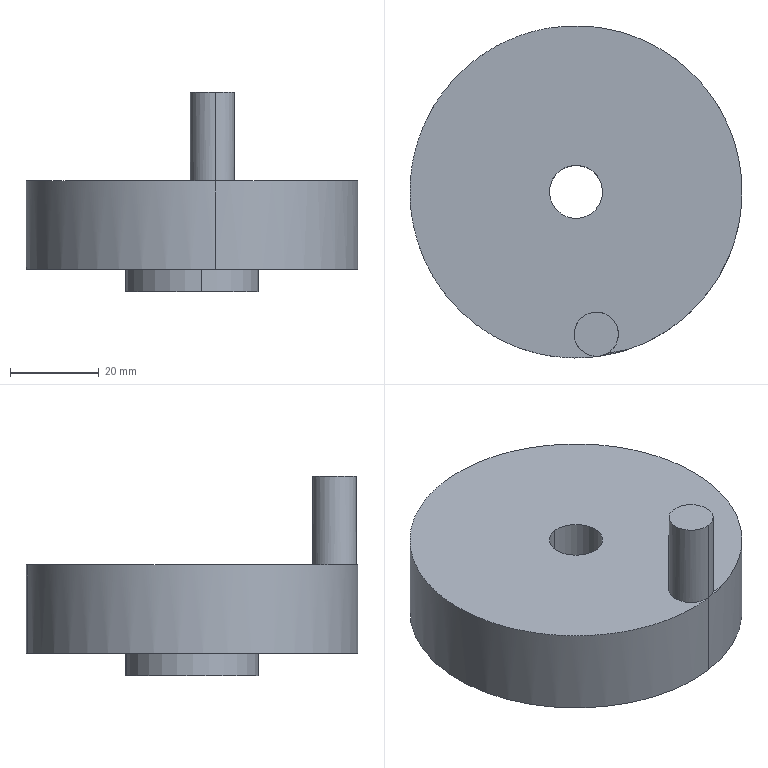Component | SolidWorks | Turntable-2 | 1 solid | 12 faces | box 75 x 75 x 45 mm | volume 90635 mm3 | cylinder 8 | plane 4 | commonest cylinder face diameters 30 x2 10 x2 12 x2 75 x2
build123d program:
from build123d import *

# Parameters (mm, degrees)
SKETCH1_R           = 37.5
SKETCH1_R_2         = 6
BOSS_EXTRUDE1_DEPTH = 20
SKETCH2_R           = 5
BOSS_EXTRUDE2_DEPTH = 20
SKETCH3_R           = 15
SKETCH3_R_2         = 6
BOSS_EXTRUDE3_DEPTH = 5


with BuildPart() as part:
    # Sketch1 → Boss-Extrude1 (new body)
    with BuildSketch(Plane.XY):
        with Locations((-30, 0)):
            Circle(SKETCH1_R)
        with Locations((-30, 0)):
            Circle(SKETCH1_R_2, mode=Mode.SUBTRACT)
    extrude(amount=-BOSS_EXTRUDE1_DEPTH)

    # Sketch2 → Boss-Extrude2 (add)
    with BuildSketch(Plane.XY):
        with Locations((2.5, 0)):
            Circle(SKETCH2_R)
    extrude(amount=BOSS_EXTRUDE2_DEPTH)

    # Sketch3 → Boss-Extrude3 (add)
    with BuildSketch(Plane(origin=(0, 0, -20), x_dir=(-1, 0, 0), z_dir=(0, 0, -1))):
        with Locations(Location((30, 0, 0), (0, 0, 180))):
            Circle(SKETCH3_R)
        with Locations(Location((30, 0, 0), (0, 0, 180))):
            Circle(SKETCH3_R_2, mode=Mode.SUBTRACT)
    extrude(amount=BOSS_EXTRUDE3_DEPTH)


solid = part.part

# Placed as in the assembly
solid = solid.moved(Location((-65.143, -96.872, 127.182), (0, 0, -81.89)))
STEP:
#1=COLOUR_RGB('',0.7922,0.8196,0.9333);
#2=FILL_AREA_STYLE_COLOUR('',#1);
#3=FILL_AREA_STYLE('',(#2));
#4=SURFACE_STYLE_FILL_AREA(#3);
#5=SURFACE_SIDE_STYLE('',(#4));
#6=SURFACE_STYLE_USAGE(.BOTH.,#5);
#7=PRESENTATION_STYLE_ASSIGNMENT((#6));
#8=CARTESIAN_POINT('',(-2.815,-2.06,4.023));
#9=VERTEX_POINT('',#8);
#10=CARTESIAN_POINT('',(-2.648,-3.229,4.023));
#11=VERTEX_POINT('',#10);
#12=CARTESIAN_POINT('',(-2.731,-2.645,4.023));
#13=DIRECTION('',(0.,-0.,-1.));
#14=DIRECTION('',(-0.1411,0.99,0.));
#15=AXIS2_PLACEMENT_3D('',#12,#13,#14);
#16=CIRCLE('',#15,0.5906);
#17=EDGE_CURVE('',#9,#11,#16,.T.);
#18=ORIENTED_EDGE('',*,*,#17,.F.);
#19=CARTESIAN_POINT('',(-2.815,-2.06,4.22));
#20=VERTEX_POINT('',#19);
#21=CARTESIAN_POINT('',(-2.815,-2.06,4.023));
#22=DIRECTION('',(-0.,0.,1.));
#23=VECTOR('',#22,39.37);
#24=LINE('',#21,#23);
#25=EDGE_CURVE('',#9,#20,#24,.T.);
#26=ORIENTED_EDGE('',*,*,#25,.T.);
#27=CARTESIAN_POINT('',(-2.648,-3.229,4.22));
#28=VERTEX_POINT('',#27);
#29=CARTESIAN_POINT('',(-2.731,-2.645,4.22));
#30=DIRECTION('',(0.,-0.,-1.));
#31=DIRECTION('',(0.1411,-0.99,0.));
#32=AXIS2_PLACEMENT_3D('',#29,#30,#31);
#33=CIRCLE('',#32,0.5906);
#34=EDGE_CURVE('',#20,#28,#33,.T.);
#35=ORIENTED_EDGE('',*,*,#34,.T.);
#36=CARTESIAN_POINT('',(-2.648,-3.229,4.023));
#37=DIRECTION('',(-0.,0.,1.));
#38=VECTOR('',#37,39.37);
#39=LINE('',#36,#38);
#40=EDGE_CURVE('',#11,#28,#39,.T.);
#41=ORIENTED_EDGE('',*,*,#40,.F.);
#42=EDGE_LOOP('',(#18,#26,#35,#41));
#43=FACE_OUTER_BOUND('',#42,.T.);
#44=CARTESIAN_POINT('',(-2.731,-2.645,4.023));
#45=DIRECTION('',(-0.,0.,1.));
#46=DIRECTION('',(0.1411,-0.99,0.));
#47=AXIS2_PLACEMENT_3D('',#44,#45,#46);
#48=CYLINDRICAL_SURFACE('',#47,0.5906);
#49=ADVANCED_FACE('',(#43),#48,.T.);
#50=CARTESIAN_POINT('',(-2.523,-4.106,5.795));
#51=VERTEX_POINT('',#50);
#52=CARTESIAN_POINT('',(-2.579,-3.716,5.795));
#53=VERTEX_POINT('',#52);
#54=CARTESIAN_POINT('',(-2.551,-3.911,5.795));
#55=DIRECTION('',(-0.,0.,1.));
#56=DIRECTION('',(0.1411,-0.99,0.));
#57=AXIS2_PLACEMENT_3D('',#54,#55,#56);
#58=CIRCLE('',#57,0.1969);
#59=EDGE_CURVE('',#51,#53,#58,.T.);
#60=ORIENTED_EDGE('',*,*,#59,.F.);
#61=CARTESIAN_POINT('',(-2.523,-4.106,5.007));
#62=VERTEX_POINT('',#61);
#63=CARTESIAN_POINT('',(-2.523,-4.106,5.795));
#64=DIRECTION('',(0.,-0.,-1.));
#65=VECTOR('',#64,39.37);
#66=LINE('',#63,#65);
#67=EDGE_CURVE('',#51,#62,#66,.T.);
#68=ORIENTED_EDGE('',*,*,#67,.T.);
#69=CARTESIAN_POINT('',(-2.579,-3.716,5.007));
#70=VERTEX_POINT('',#69);
#71=CARTESIAN_POINT('',(-2.551,-3.911,5.007));
#72=DIRECTION('',(-0.,0.,1.));
#73=DIRECTION('',(0.1411,-0.99,0.));
#74=AXIS2_PLACEMENT_3D('',#71,#72,#73);
#75=CIRCLE('',#74,0.1969);
#76=EDGE_CURVE('',#62,#70,#75,.T.);
#77=ORIENTED_EDGE('',*,*,#76,.T.);
#78=CARTESIAN_POINT('',(-2.579,-3.716,5.795));
#79=DIRECTION('',(0.,-0.,-1.));
#80=VECTOR('',#79,39.37);
#81=LINE('',#78,#80);
#82=EDGE_CURVE('',#53,#70,#81,.T.);
#83=ORIENTED_EDGE('',*,*,#82,.F.);
#84=EDGE_LOOP('',(#60,#68,#77,#83));
#85=FACE_OUTER_BOUND('',#84,.T.);
#86=CARTESIAN_POINT('',(-2.551,-3.911,5.795));
#87=DIRECTION('',(0.,-0.,-1.));
#88=DIRECTION('',(-0.1411,0.99,0.));
#89=AXIS2_PLACEMENT_3D('',#86,#87,#88);
#90=CYLINDRICAL_SURFACE('',#89,0.1969);
#91=ADVANCED_FACE('',(#85),#90,.T.);
#92=CARTESIAN_POINT('',(-2.698,-2.878,4.023));
#93=VERTEX_POINT('',#92);
#94=CARTESIAN_POINT('',(-2.765,-2.411,4.023));
#95=VERTEX_POINT('',#94);
#96=CARTESIAN_POINT('',(-2.731,-2.645,4.023));
#97=DIRECTION('',(0.,-0.,-1.));
#98=DIRECTION('',(-0.1411,0.99,0.));
#99=AXIS2_PLACEMENT_3D('',#96,#97,#98);
#100=CIRCLE('',#99,0.2362);
#101=EDGE_CURVE('',#93,#95,#100,.T.);
#102=ORIENTED_EDGE('',*,*,#101,.T.);
#103=CARTESIAN_POINT('',(-2.765,-2.411,5.007));
#104=VERTEX_POINT('',#103);
#105=CARTESIAN_POINT('',(-2.765,-2.411,4.22));
#106=DIRECTION('',(-0.,0.,1.));
#107=VECTOR('',#106,39.37);
#108=LINE('',#105,#107);
#109=EDGE_CURVE('',#95,#104,#108,.T.);
#110=ORIENTED_EDGE('',*,*,#109,.T.);
#111=CARTESIAN_POINT('',(-2.698,-2.878,5.007));
#112=VERTEX_POINT('',#111);
#113=CARTESIAN_POINT('',(-2.731,-2.645,5.007));
#114=DIRECTION('',(-0.,0.,1.));
#115=DIRECTION('',(0.1411,-0.99,0.));
#116=AXIS2_PLACEMENT_3D('',#113,#114,#115);
#117=CIRCLE('',#116,0.2362);
#118=EDGE_CURVE('',#104,#112,#117,.T.);
#119=ORIENTED_EDGE('',*,*,#118,.T.);
#120=CARTESIAN_POINT('',(-2.698,-2.878,4.22));
#121=DIRECTION('',(-0.,0.,1.));
#122=VECTOR('',#121,39.37);
#123=LINE('',#120,#122);
#124=EDGE_CURVE('',#93,#112,#123,.T.);
#125=ORIENTED_EDGE('',*,*,#124,.F.);
#126=EDGE_LOOP('',(#102,#110,#119,#125));
#127=FACE_OUTER_BOUND('',#126,.T.);
#128=CARTESIAN_POINT('',(-2.731,-2.645,4.22));
#129=DIRECTION('',(-0.,0.,1.));
#130=DIRECTION('',(0.1411,-0.99,0.));
#131=AXIS2_PLACEMENT_3D('',#128,#129,#130);
#132=CYLINDRICAL_SURFACE('',#131,0.2362);
#133=ADVANCED_FACE('',(#127),#132,.F.);
#134=CARTESIAN_POINT('',(-2.523,-4.106,4.22));
#135=VERTEX_POINT('',#134);
#136=CARTESIAN_POINT('',(-2.94,-1.183,4.22));
#137=VERTEX_POINT('',#136);
#138=CARTESIAN_POINT('',(-2.731,-2.645,4.22));
#139=DIRECTION('',(-0.,0.,1.));
#140=DIRECTION('',(0.1411,-0.99,0.));
#141=AXIS2_PLACEMENT_3D('',#138,#139,#140);
#142=CIRCLE('',#141,1.476);
#143=EDGE_CURVE('',#135,#137,#142,.T.);
#144=ORIENTED_EDGE('',*,*,#143,.T.);
#145=CARTESIAN_POINT('',(-2.94,-1.183,5.007));
#146=VERTEX_POINT('',#145);
#147=CARTESIAN_POINT('',(-2.94,-1.183,4.22));
#148=DIRECTION('',(-0.,0.,1.));
#149=VECTOR('',#148,39.37);
#150=LINE('',#147,#149);
#151=EDGE_CURVE('',#137,#146,#150,.T.);
#152=ORIENTED_EDGE('',*,*,#151,.T.);
#153=CARTESIAN_POINT('',(-2.731,-2.645,5.007));
#154=DIRECTION('',(-0.,0.,1.));
#155=DIRECTION('',(0.1411,-0.99,0.));
#156=AXIS2_PLACEMENT_3D('',#153,#154,#155);
#157=CIRCLE('',#156,1.476);
#158=EDGE_CURVE('',#62,#146,#157,.T.);
#159=ORIENTED_EDGE('',*,*,#158,.F.);
#160=CARTESIAN_POINT('',(-2.523,-4.106,4.22));
#161=DIRECTION('',(-0.,0.,1.));
#162=VECTOR('',#161,39.37);
#163=LINE('',#160,#162);
#164=EDGE_CURVE('',#135,#62,#163,.T.);
#165=ORIENTED_EDGE('',*,*,#164,.F.);
#166=EDGE_LOOP('',(#144,#152,#159,#165));
#167=FACE_OUTER_BOUND('',#166,.T.);
#168=CARTESIAN_POINT('',(-2.731,-2.645,4.22));
#169=DIRECTION('',(-0.,0.,1.));
#170=DIRECTION('',(0.1411,-0.99,0.));
#171=AXIS2_PLACEMENT_3D('',#168,#169,#170);
#172=CYLINDRICAL_SURFACE('',#171,1.476);
#173=ADVANCED_FACE('',(#167),#172,.T.);
#174=ORIENTED_EDGE('',*,*,#143,.F.);
#175=CARTESIAN_POINT('',(-2.731,-2.645,4.22));
#176=DIRECTION('',(-0.,0.,1.));
#177=DIRECTION('',(0.1411,-0.99,0.));
#178=AXIS2_PLACEMENT_3D('',#175,#176,#177);
#179=CIRCLE('',#178,1.476);
#180=EDGE_CURVE('',#137,#135,#179,.T.);
#181=ORIENTED_EDGE('',*,*,#180,.F.);
#182=EDGE_LOOP('',(#174,#181));
#183=FACE_OUTER_BOUND('',#182,.T.);
#184=CARTESIAN_POINT('',(-2.731,-2.645,4.22));
#185=DIRECTION('',(0.,-0.,-1.));
#186=DIRECTION('',(0.1411,-0.99,0.));
#187=AXIS2_PLACEMENT_3D('',#184,#185,#186);
#188=CIRCLE('',#187,0.5906);
#189=EDGE_CURVE('',#28,#20,#188,.T.);
#190=ORIENTED_EDGE('',*,*,#189,.F.);
#191=ORIENTED_EDGE('',*,*,#34,.F.);
#192=EDGE_LOOP('',(#190,#191));
#193=FACE_BOUND('',#192,.T.);
#194=CARTESIAN_POINT('',(-2.731,-2.645,4.22));
#195=DIRECTION('',(-0.,0.,1.));
#196=DIRECTION('',(0.1411,-0.99,0.));
#197=AXIS2_PLACEMENT_3D('',#194,#195,#196);
#198=PLANE('',#197);
#199=ADVANCED_FACE('',(#183,#193),#198,.F.);
#200=ORIENTED_EDGE('',*,*,#151,.F.);
#201=ORIENTED_EDGE('',*,*,#180,.T.);
#202=ORIENTED_EDGE('',*,*,#164,.T.);
#203=CARTESIAN_POINT('',(-2.731,-2.645,5.007));
#204=DIRECTION('',(-0.,0.,1.));
#205=DIRECTION('',(0.1411,-0.99,0.));
#206=AXIS2_PLACEMENT_3D('',#203,#204,#205);
#207=CIRCLE('',#206,1.476);
#208=EDGE_CURVE('',#146,#62,#207,.T.);
#209=ORIENTED_EDGE('',*,*,#208,.F.);
#210=EDGE_LOOP('',(#200,#201,#202,#209));
#211=FACE_OUTER_BOUND('',#210,.T.);
#212=CARTESIAN_POINT('',(-2.731,-2.645,4.22));
#213=DIRECTION('',(-0.,0.,1.));
#214=DIRECTION('',(0.1411,-0.99,0.));
#215=AXIS2_PLACEMENT_3D('',#212,#213,#214);
#216=CYLINDRICAL_SURFACE('',#215,1.476);
#217=ADVANCED_FACE('',(#211),#216,.T.);
#218=CARTESIAN_POINT('',(-2.731,-2.645,5.007));
#219=DIRECTION('',(-0.,0.,1.));
#220=DIRECTION('',(0.1411,-0.99,0.));
#221=AXIS2_PLACEMENT_3D('',#218,#219,#220);
#222=CIRCLE('',#221,0.2362);
#223=EDGE_CURVE('',#112,#104,#222,.T.);
#224=ORIENTED_EDGE('',*,*,#223,.F.);
#225=ORIENTED_EDGE('',*,*,#118,.F.);
#226=EDGE_LOOP('',(#224,#225));
#227=FACE_BOUND('',#226,.T.);
#228=ORIENTED_EDGE('',*,*,#158,.T.);
#229=ORIENTED_EDGE('',*,*,#208,.T.);
#230=CARTESIAN_POINT('',(-2.551,-3.911,5.007));
#231=DIRECTION('',(-0.,0.,1.));
#232=DIRECTION('',(0.1411,-0.99,0.));
#233=AXIS2_PLACEMENT_3D('',#230,#231,#232);
#234=CIRCLE('',#233,0.1969);
#235=EDGE_CURVE('',#70,#62,#234,.T.);
#236=ORIENTED_EDGE('',*,*,#235,.F.);
#237=ORIENTED_EDGE('',*,*,#76,.F.);
#238=EDGE_LOOP('',(#228,#229,#236,#237));
#239=FACE_OUTER_BOUND('',#238,.T.);
#240=CARTESIAN_POINT('',(-2.731,-2.645,5.007));
#241=DIRECTION('',(-0.,0.,1.));
#242=DIRECTION('',(0.1411,-0.99,0.));
#243=AXIS2_PLACEMENT_3D('',#240,#241,#242);
#244=PLANE('',#243);
#245=ADVANCED_FACE('',(#227,#239),#244,.T.);
#246=ORIENTED_EDGE('',*,*,#109,.F.);
#247=CARTESIAN_POINT('',(-2.731,-2.645,4.023));
#248=DIRECTION('',(0.,-0.,-1.));
#249=DIRECTION('',(-0.1411,0.99,0.));
#250=AXIS2_PLACEMENT_3D('',#247,#248,#249);
#251=CIRCLE('',#250,0.2362);
#252=EDGE_CURVE('',#95,#93,#251,.T.);
#253=ORIENTED_EDGE('',*,*,#252,.T.);
#254=ORIENTED_EDGE('',*,*,#124,.T.);
#255=ORIENTED_EDGE('',*,*,#223,.T.);
#256=EDGE_LOOP('',(#246,#253,#254,#255));
#257=FACE_OUTER_BOUND('',#256,.T.);
#258=CARTESIAN_POINT('',(-2.731,-2.645,4.22));
#259=DIRECTION('',(-0.,0.,1.));
#260=DIRECTION('',(0.1411,-0.99,0.));
#261=AXIS2_PLACEMENT_3D('',#258,#259,#260);
#262=CYLINDRICAL_SURFACE('',#261,0.2362);
#263=ADVANCED_FACE('',(#257),#262,.F.);
#264=ORIENTED_EDGE('',*,*,#67,.F.);
#265=CARTESIAN_POINT('',(-2.551,-3.911,5.795));
#266=DIRECTION('',(-0.,0.,1.));
#267=DIRECTION('',(0.1411,-0.99,0.));
#268=AXIS2_PLACEMENT_3D('',#265,#266,#267);
#269=CIRCLE('',#268,0.1969);
#270=EDGE_CURVE('',#53,#51,#269,.T.);
#271=ORIENTED_EDGE('',*,*,#270,.F.);
#272=ORIENTED_EDGE('',*,*,#82,.T.);
#273=ORIENTED_EDGE('',*,*,#235,.T.);
#274=EDGE_LOOP('',(#264,#271,#272,#273));
#275=FACE_OUTER_BOUND('',#274,.T.);
#276=CARTESIAN_POINT('',(-2.551,-3.911,5.795));
#277=DIRECTION('',(0.,-0.,-1.));
#278=DIRECTION('',(-0.1411,0.99,0.));
#279=AXIS2_PLACEMENT_3D('',#276,#277,#278);
#280=CYLINDRICAL_SURFACE('',#279,0.1969);
#281=ADVANCED_FACE('',(#275),#280,.T.);
#282=ORIENTED_EDGE('',*,*,#270,.T.);
#283=ORIENTED_EDGE('',*,*,#59,.T.);
#284=EDGE_LOOP('',(#282,#283));
#285=FACE_OUTER_BOUND('',#284,.T.);
#286=CARTESIAN_POINT('',(-2.551,-3.911,5.795));
#287=DIRECTION('',(-0.,0.,1.));
#288=DIRECTION('',(0.1411,-0.99,0.));
#289=AXIS2_PLACEMENT_3D('',#286,#287,#288);
#290=PLANE('',#289);
#291=ADVANCED_FACE('',(#285),#290,.T.);
#292=CARTESIAN_POINT('',(-2.731,-2.645,4.023));
#293=DIRECTION('',(0.,-0.,-1.));
#294=DIRECTION('',(-0.1411,0.99,0.));
#295=AXIS2_PLACEMENT_3D('',#292,#293,#294);
#296=CIRCLE('',#295,0.5906);
#297=EDGE_CURVE('',#11,#9,#296,.T.);
#298=ORIENTED_EDGE('',*,*,#297,.T.);
#299=ORIENTED_EDGE('',*,*,#17,.T.);
#300=EDGE_LOOP('',(#298,#299));
#301=FACE_OUTER_BOUND('',#300,.T.);
#302=ORIENTED_EDGE('',*,*,#101,.F.);
#303=ORIENTED_EDGE('',*,*,#252,.F.);
#304=EDGE_LOOP('',(#302,#303));
#305=FACE_BOUND('',#304,.T.);
#306=CARTESIAN_POINT('',(-2.731,-2.645,4.023));
#307=DIRECTION('',(0.,-0.,-1.));
#308=DIRECTION('',(-0.1411,0.99,-0.));
#309=AXIS2_PLACEMENT_3D('',#306,#307,#308);
#310=PLANE('',#309);
#311=ADVANCED_FACE('',(#301,#305),#310,.T.);
#312=ORIENTED_EDGE('',*,*,#25,.F.);
#313=ORIENTED_EDGE('',*,*,#297,.F.);
#314=ORIENTED_EDGE('',*,*,#40,.T.);
#315=ORIENTED_EDGE('',*,*,#189,.T.);
#316=EDGE_LOOP('',(#312,#313,#314,#315));
#317=FACE_OUTER_BOUND('',#316,.T.);
#318=CARTESIAN_POINT('',(-2.731,-2.645,4.023));
#319=DIRECTION('',(-0.,0.,1.));
#320=DIRECTION('',(0.1411,-0.99,0.));
#321=AXIS2_PLACEMENT_3D('',#318,#319,#320);
#322=CYLINDRICAL_SURFACE('',#321,0.5906);
#323=ADVANCED_FACE('',(#317),#322,.T.);
#324=CLOSED_SHELL('',(#49,#91,#133,#173,#199,#217,#245,#263,#281,#291,#311,#323));
#325=MANIFOLD_SOLID_BREP('',#324);
#326=STYLED_ITEM('',(#7),#325);
#327=PRESENTATION_LAYER_ASSIGNMENT('','',(#326));
#328=(LENGTH_UNIT()NAMED_UNIT(*)SI_UNIT($,.METRE.));
#329=LENGTH_MEASURE_WITH_UNIT(LENGTH_MEASURE(0.0254),#328);
#330=DIMENSIONAL_EXPONENTS(1.,0.,0.,0.,0.,0.,0.);
#331=(CONVERSION_BASED_UNIT('',#329)LENGTH_UNIT()NAMED_UNIT(#330));
#332=UNCERTAINTY_MEASURE_WITH_UNIT(LENGTH_MEASURE(0.00001),#331,'','');
#333=(NAMED_UNIT(*)PLANE_ANGLE_UNIT()SI_UNIT($,.RADIAN.));
#334=(NAMED_UNIT(*)SI_UNIT($,.STERADIAN.)SOLID_ANGLE_UNIT());
#335=(GEOMETRIC_REPRESENTATION_CONTEXT(3)GLOBAL_UNCERTAINTY_ASSIGNED_CONTEXT((#332))GLOBAL_UNIT_ASSIGNED_CONTEXT((#331,#333,#334))REPRESENTATION_CONTEXT('',''));
#336=MECHANICAL_DESIGN_GEOMETRIC_PRESENTATION_REPRESENTATION('',(#326),#335);
#337=CARTESIAN_POINT('',(0.,0.,0.));
#338=DIRECTION('',(0.,0.,1.));
#339=DIRECTION('',(1.,0.,0.));
#340=AXIS2_PLACEMENT_3D('',#337,#338,#339);
#341=(LENGTH_UNIT()NAMED_UNIT(*)SI_UNIT($,.METRE.));
#342=LENGTH_MEASURE_WITH_UNIT(LENGTH_MEASURE(0.0254),#341);
#343=DIMENSIONAL_EXPONENTS(1.,0.,0.,0.,0.,0.,0.);
#344=(CONVERSION_BASED_UNIT('',#342)LENGTH_UNIT()NAMED_UNIT(#343));
#345=UNCERTAINTY_MEASURE_WITH_UNIT(LENGTH_MEASURE(0.00001),#344,'','');
#346=(NAMED_UNIT(*)PLANE_ANGLE_UNIT()SI_UNIT($,.RADIAN.));
#347=(NAMED_UNIT(*)SI_UNIT($,.STERADIAN.)SOLID_ANGLE_UNIT());
#348=(GEOMETRIC_REPRESENTATION_CONTEXT(3)GLOBAL_UNCERTAINTY_ASSIGNED_CONTEXT((#345))GLOBAL_UNIT_ASSIGNED_CONTEXT((#344,#346,#347))REPRESENTATION_CONTEXT('',''));
#349=ADVANCED_BREP_SHAPE_REPRESENTATION('',(#325,#340),#348);